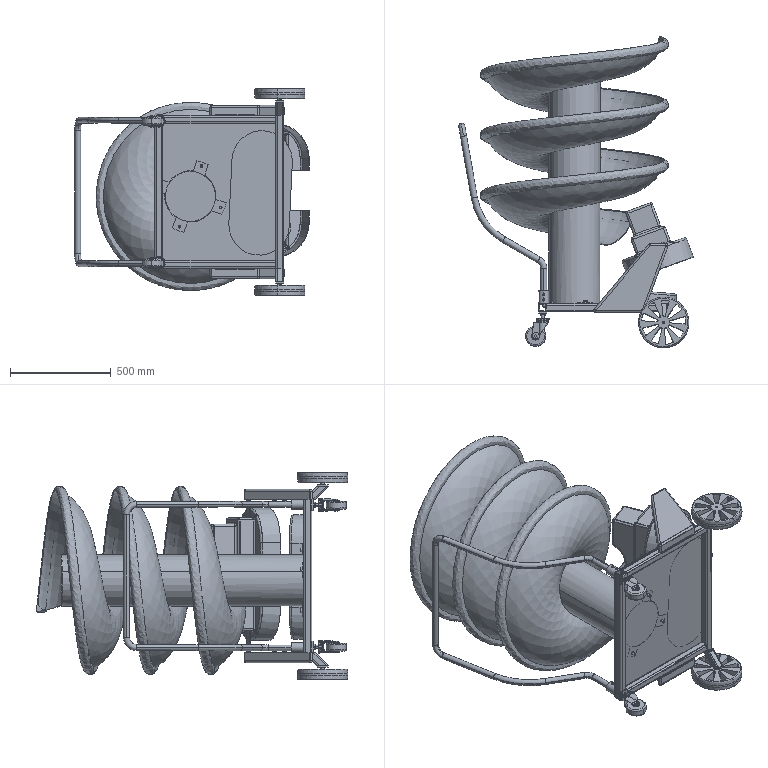Assembly | SolidWorks | mm | 43 component files | 46 solids | 1810 faces | box 1163.5 x 1546.21 x 1026 mm | volume 42101622 mm3 | cylinder 650 | plane 611 | sphere 176 | cone 160 | torus 140 | spline 73 | commonest cylinder face diameters 6 x106 20 x60 16 x50 12 x32 10 x32 14 x28 8 x24 60 x24
Bill of materials:
01-01-01ChassisWeldment1 | 1 | Q235 | Flat rectangular open frame made of four straight hollow rectangular-section tube members: two longer uprights with two shorter cross members fitted between them at the ends.
01-01-02ChassisWeldment2 | 2 | Q235 | Short length of hollow rectangular tube with rounded outer and inner corners. One end appears cut square and the other at an angle.
01-01-03ChassisWeldment3 | 2 | Q235 | Thick flat rectangular plate with rounded corners and one plain round through-hole, offset from the plate center.
01-01-04ChassisWeldment4 | 1 | Q235 | Thin flat rectangular sheet panel with four small round through-holes, spaced irregularly across the face.
01-01-05ChassisWeldment5 | 2 | 45 | Thick-walled cylindrical sleeve (bushing-like tube) with a large central bore and two small radial holes in a line along one side.
01-02WheelAxis | 2 | 45 | Stepped turned cylindrical part with a central axial bore and three diameters: a middle collar (largest), a longer upper section and a smaller lower spigot, with small chamfers at the ends.
01-03Wheel | 2 | RubberⅠ- 2 | Short disc or wheel-shaped part with a rounded outer rim, ten wedge-shaped radial cutouts forming spokes, and a small central hole.
01-04RearWheelConnectionPlate | 2 | Q235 | Flat rectangular plate with rounded corners and one round through-hole, offset toward one end.
02-01RollingTrack | 1 |  | Screw auger or helical flight: a hollow cylindrical central shaft carrying about three turns of a dished helical flight with a rolled or beaded outer edge, and small tabbed flanges with holes at one shaft end.
02-02Handrail | 1 |  | Bent round rod or tube formed into a three-dimensional U-shaped loop, with two parallel legs that each have offset joggle bends near their open ends.
03-01MotorBracket1 | 2 |  | Thin flat plate with an irregular tapered quadrilateral or pentagonal outline: a wide base edge tapering to a narrow, angled tip with a short chamfered corner.
03-02MotorBracket1 | 1 | Q235 | Long narrow flat strip with two wider square pad regions along its length. Each pad has a central round hole and four small corner holes.
03-03BallDeliveryWheel | 2 |  | Plain short solid cylinder (disc/slug) with flat parallel end faces; length is less than the diameter.
04-01MotorBracketHousing | 1 |  | Thin, flat trapezoidal plate or lid with rounded corners and edges, a solid closed top face, and several small rectangular tabs sticking out from the underside along the edges.
04-02Housing | 1 |  | Thin-walled stadium-shaped (obround) band with large rectangular gaps cut through both long sides. A stepped rectangular block projects from one side of the band, and this block has a semicircular notch cut into one edge.
04-03BottomHousing | 1 |  | Thin, flat stadium-shaped (obround) plate with a small notch in the middle of one long edge.
AC1-08M30HC0A1 | 2 |  | Box-shaped body with a square front flange, four corner through-holes, a raised circular boss in the centre of the flange, and a protruding cylindrical shaft with a flat on it. Long steps or grooves run the length of the body, and a narrower rectangular block sits at the rear. The overall shape looks like an electric motor body.
Caster-WHB31-D100-P | 2 |  | Swivel-caster-like assembly: a cylindrical wheel held in a curved single-sided fork, an axle hub with a hex nut, a round flange or washer stack on top, and a plain cylindrical stem pin pointing up.
GB_T276-94DeepGrooveBallBearing6202 | 2 | GCr4 | Open radial ball-bearing-like assembly: concentric outer and inner rings with eight spherical balls in the gap between them. No cage or shields are visible.
GB_T5781-2000HexHeadBoltFullThreadCM12x25 | 4 | 3.6 Grade | Hex-head bolt with a washer face under the head, a plain cylindrical shank and a chamfered tip.
GB_T6172.1-2000HexThinNutAAndBM16 | 2 | 04 Grade | Thin hexagonal nut with a plain cylindrical through-bore and chamfered corners on both faces.
GB_T70.1-2000_SocketHeadCapScrew_M6_16 | 2 | 8.8 Grade | Socket-head cap screw shape: a cylindrical head with a hexagonal recess, a plain cylindrical shank and a chamfered tip.
GB73-85SlottedFlatPointSetScrewM10x12 | 4 | 14H Grade | Short headless cylindrical pin with a straight slot across one end face, a small chamfer on the slotted end and a larger chamfer at the other end, similar to a slotted set screw.
Mirror04-01MotorBracketHousing | 1 |  | Shallow, open, thin-walled trapezoidal tray with rounded corners, a flat floor and small rectangular tabs standing up along the top rim.
Mates:
1. concentric | 01-02WheelAxis-1 face at (300, -53.25, 474) dir (0, 0, 1) r 6 | 01-01Chassis-1/01-01-03ChassisWeldment3-1 face at (300, -53.25, 453) dir (0, 0, 1) r 6
2. coincident | 01-01Chassis-1/01-01-03ChassisWeldment3-1 face at (314, -31.5, 453) dir (0, 0, 1) | 01-02WheelAxis-1 face at (300, -53.25, 453) dir (0, 0, -1)
3. coincident | 01-01Chassis-1 plane at (0, 0, 0) dir (0, 1, 0) | assembly plane at (0, 0, 0) dir (0, 1, 0)
4. coincident | 01-01Chassis-1 plane at (0, 0, 0) dir (0, 0, 1) | assembly plane at (0, 0, 0) dir (0, 0, 1)
5. coincident | 01-01Chassis-1 plane at (0, 0, 0) dir (1, 0, 0) | assembly plane at (0, 0, 0) dir (1, 0, 0)
6. concentric | 01-02WheelAxis-1 face at (300, -53.25, 474) dir (0, 0, 1) r 7.5 | GB_T276-94DeepGrooveBallBearing6202-2 face at (300, -53.25, 456.079) dir (0, 0, -1) r 7.5
7. coincident | 01-02WheelAxis-1 face at (300, -53.25, 463) dir (0, 0, 1) | GB_T276-94DeepGrooveBallBearing6202-2 face at (300, -42.45, 463) dir (0, 0, -1)
8. concentric | GB_T276-94DeepGrooveBallBearing6202-2 face at (300, -53.25, 468.5) dir (0, 0, -1) r 17.5 | 01-03Wheel-1 face at (300, -53.25, 474) dir (0, 0, -1) r 17.5
9. coincident | GB_T276-94DeepGrooveBallBearing6202-2 face at (300, -42.45, 474) dir (0, 0, 1) | 01-03Wheel-1 face at (300, -53.25, 474) dir (0, 0, -1)
10. concentric | 01-02WheelAxis-1 face at (300, -53.25, 474) dir (0, 0, 1) r 3 | GB_T70.1-2000_SocketHeadCapScrew_M6_16-1 face at (300, -53.25, 489) dir (0, 0, 1) r 3
11. coincident | 01-03Wheel-1 edge at (300, -53.25, 483) dir (0, 0, 1) r 4.5 | GB_T70.1-2000_SocketHeadCapScrew_M6_16-1 face at (300.832, -48.32, 483) dir (0, 0, -1)
12. coincident | 01-01Chassis-1/01-01-01ChassisWeldment1-1 face at (-312, 0, 360) dir (0, -1, 0) | 01-04RearWheelConnectionPlate-1 face at (-286, 0, 330.5) dir (0, 1, 0)
13. coincident | 01-01Chassis-1/01-01-01ChassisWeldment1-1 face at (-300, 40, 380) dir (0, 0, 1) | 01-04RearWheelConnectionPlate-1 face at (-314, 0, 380) dir (0, 0, 1)
14. coincident | 01-01Chassis-1/01-01-01ChassisWeldment1-1 face at (-320, 8, 360) dir (-1, 0, 0) | 01-04RearWheelConnectionPlate-1 face at (-320, 0, 330.5) dir (-1, 0, 0)
15. concentric | Caster-WHB31-D100-P-1 face at (-300, -171, 352.25) dir (0, -1, 0) r 8 | 01-04RearWheelConnectionPlate-1 face at (-300, 0, 352.25) dir (0, 1, 0) r 7
16. coincident | Caster-WHB31-D100-P-1 face at (-306.582, 0, 345.111) dir (0, 1, 0) | 01-04RearWheelConnectionPlate-1 face at (-286, 0, 330.5) dir (0, 1, 0)
17. concentric | Caster-WHB31-D100-P-1 face at (-300, -171, 352.25) dir (0, -1, 0) r 8 | GB_T6172.1-2000HexThinNutAAndBM16-1 face at (-300, -16, 352.25) dir (0, 1, 0) r 8
18. coincident | 01-04RearWheelConnectionPlate-1 face at (-286, -8, 330.5) dir (0, -1, 0) | GB_T6172.1-2000HexThinNutAAndBM16-1 face at (-276.834, -8, 352.25) dir (0, 1, 0)
19. parallel | 01-04RearWheelConnectionPlate-1 face at (-320, 0, 330.5) dir (-1, 0, 0) | GB_T6172.1-2000HexThinNutAAndBM16-1 face at (-311.583, -16, 358.938) dir (-1, 0, 0)
20. coincident | 01-01Chassis-1/01-01-04ChassisWeldment4-1 face at (-315, 43, 375) dir (0, 1, 0) | 02-01RollingTrack-1 face at (-142.96, 43, -22.04) dir (0, -1, 0)
21. angle | 01-01Chassis-1/01-01-01ChassisWeldment1-1 face at (300, 8, 380) dir (0, 0, 1) | 02-01RollingTrack-1 face at (-132.7, 48, 6.151) dir (0.342, 0, 0.9397)
22. coincident | 01-01Chassis-1/01-01-01ChassisWeldment1-1 face at (300, 0, 372) dir (0, -1, 0) | 03-01MotorBracket1-1 face at (-24.135, 0, 380) dir (0, -1, 0)
23. concentric | 01-01Chassis-1/01-01-05ChassisWeldment5-1 face at (-295, 103, 355) dir (0, -1, 0) r 15.1 | 02-02Handrail-1 face at (-295, 43, 355) dir (0, 1, 0) r 15
24. concentric | 01-01Chassis-1/01-01-05ChassisWeldment5-2 face at (-295, 103, -355) dir (0, -1, 0) r 15.1 | 02-02Handrail-1 face at (-295, 214.132, -355) dir (0, -1, 0) r 15
25. coincident | 01-01Chassis-1/01-01-04ChassisWeldment4-1 face at (-315, 43, 375) dir (0, 1, 0) | 02-02Handrail-1 face at (-295, 43, 355) dir (0, -1, 0)
26. concentric | 01-01Chassis-1/01-01-05ChassisWeldment5-1 face at (-295, 84, 355) dir (0, 0, -1) r 5 | GB73-85SlottedFlatPointSetScrewM10x12-1 face at (-295, 84, 382.55) dir (0, 0, 1) r 5
27. tangent | 02-02Handrail-1 face at (-295, 43, 355) dir (0, 1, 0) r 15 | GB73-85SlottedFlatPointSetScrewM10x12-1 face at (-295, 84, 370) dir (0, 0, -1)
28. coincident | 01-01Chassis-1/01-01-01ChassisWeldment1-1 face at (300, 8, 380) dir (0, 0, 1) | 03-01MotorBracket1-1 face at (-24.135, 0, 380) dir (0, 0, -1)
29. coincident | 03-01MotorBracket1-1 face at (-92.322, 187.34, 374) dir (-0.342, 0.9397, 0) | 03-02MotorBracket1-1 face at (251.015, 312.305, -1) dir (0.342, -0.9397, 0)
30. coincident | 03-01MotorBracket1-1 face at (-24.135, 0, 384) dir (0, 0, 1) | 03-02MotorBracket1-1 face at (234.57, 306.319, 384) dir (0, 0, 1)
31. coincident | 03-01MotorBracket1-1 edge at (272.158, 320, 382) dir (1, 0, 0) | 03-02MotorBracket1-1 face at (272.158, 320, 379) dir (0.9397, 0.342, 0)
32. concentric | 03-02MotorBracket1-1 face at (279.548, 326.946, 206.82) dir (-0.342, 0.9397, 0) r 2.5 | AC1-08M30HC0A1-1 face at (258.684, 384.268, 206.82) dir (-0.342, 0.9397, 0) r 3.5
33. concentric | 03-02MotorBracket1-1 face at (279.548, 326.946, 143.18) dir (-0.342, 0.9397, 0) r 2.5 | AC1-08M30HC0A1-1 face at (258.684, 384.268, 143.18) dir (-0.342, 0.9397, 0) r 3.5
34. coincident | 03-02MotorBracket1-1 face at (249.646, 316.063, -1) dir (-0.342, 0.9397, 0) | AC1-08M30HC0A1-1 face at (216.393, 303.96, 210) dir (0.342, -0.9397, 0)
35. distance | 03-03BallDeliveryWheel-1 face at (257.855, 293.511, 175) dir (-0.342, 0.9397, 0) | 03-02MotorBracket1-1 face at (251.015, 312.305, -1) dir (0.342, -0.9397, 0)
36. distance | 03-01MotorBracket1-1 edge at (-20, 4.928, 382) dir (1, 0, 0) | 01-01Chassis-1/01-01-01ChassisWeldment1-1 face at (-320, 8, 360) dir (-1, 0, 0)
37. coincident | 01-01Chassis-1/01-01-01ChassisWeldment1-1 face at (300, 8, 380) dir (0, 0, 1) | 04-01MotorBracketHousing-1 face at (-14.657, 16.888, 380) dir (0, 0, -1)
38. parallel | 03-03BallDeliveryWheel-2 face at (257.855, 293.511, -175) dir (0.342, -0.9397, 0) r 75 | 04-02Housing-1 face at (251.015, 312.305, -151.126) dir (0.342, -0.9397, 0) r 170
39. coincident | 03-02MotorBracket1-1 face at (251.015, 312.305, -1) dir (0.342, -0.9397, 0) | 04-02Housing-1 face at (251.015, 312.305, 7.874) dir (-0.342, 0.9397, 0)
40. coincident | 01-01Chassis-1/01-01-04ChassisWeldment4-1 face at (-315, 43, 375) dir (0, 1, 0) | 04-03BottomHousing-1 face at (197.547, 43, -163.468) dir (0, -1, 0)
41. coincident | 01-01Chassis-1/01-01-01ChassisWeldment1-1 face at (-320, 8, 360) dir (-1, 0, 0) | 02-01RollingTrack-1 edge at (-320, 48, 10.472) dir (0, -1, 0)
42. distance | 02-01RollingTrack-1 vertex at (-110.449, 43, 155) dir (1, 0, 0) | 01-01Chassis-1/01-01-01ChassisWeldment1-1 face at (300, 8, 380) dir (0, 0, 1)
43. concentric | 02-01RollingTrack-1 face at (-88.237, 43, 128.311) dir (0, 1, 0) r 6.75 | GB_T5781-2000HexHeadBoltFullThreadCM12x25-1 face at (-88.237, 55.5, 128.311) dir (0, 1, 0) r 6
44. coincident | 02-01RollingTrack-1 face at (-142.96, 48, -22.04) dir (0, 1, 0) | GB_T5781-2000HexHeadBoltFullThreadCM12x25-1 face at (-77.845, 48, 128.311) dir (0, -1, 0)
45. concentric | AC1-08M30HC0A1-1 face at (260.591, 285.993, 175) dir (-0.342, 0.9397, 0) r 9.5 | 03-03BallDeliveryWheel-1 face at (257.855, 293.511, 175) dir (0.342, -0.9397, 0) r 75
46. width | 04-02Housing-1 face at (208.728, 296.914, -321.126) dir (0.9397, 0.342, 0) | 04-02Housing-1 face at (293.301, 327.695, -321.126) dir (-0.9397, -0.342, 0) | 03-02MotorBracket1-1 face at (272.158, 320, 379) dir (0.9397, 0.342, 0) | 03-02MotorBracket1-1 face at (229.871, 304.609, 379) dir (-0.9397, -0.342, 0)
47. coincident | 01-01-01ChassisWeldment1-1 plane at (0, 20, 0) dir (0, 0, -1) | 01-01Chassis plane at (0, 0, 0) dir (0, 0, 1)
48. coincident | 01-01-01ChassisWeldment1-1 plane at (0, 20, 0) dir (-1, 0, 0) | 01-01Chassis plane at (0, 0, 0) dir (1, 0, 0)
49. coincident | 01-01-01ChassisWeldment1-1 face at (288, 0, 360) dir (0, -1, 0) | 01-01Chassis plane at (0, 0, 0) dir (0, 1, 0)
50. coincident | 01-01-01ChassisWeldment1-1 face at (300, 0, 380) dir (0, 0, 1) | 01-01-02ChassisWeldment2-1 face at (280, 68.222, 380) dir (0, 0, -1)
51. coincident | 01-01-01ChassisWeldment1-1 face at (312, 40, 360) dir (0, 1, 0) | 01-01-02ChassisWeldment2-1 edge at (288, 40, 380) dir (1, 0, 0)
52. coincident | 01-01-01ChassisWeldment1-1 face at (320, 32, 360) dir (1, 0, 0) | 01-01-02ChassisWeldment2-1 face at (320, 42.408, 366.279) dir (1, 0, 0)
53. coincident | 01-01-02ChassisWeldment2-1 face at (280, 68.222, 445) dir (0, 0, 1) | 01-01-03ChassisWeldment3-1 face at (314, -31.5, 445) dir (0, 0, -1)
54. distance | 01-01-03ChassisWeldment3-1 face at (286, -25.5, 453) dir (0, 1, 0) | 01-01-02ChassisWeldment2-1 edge at (312, -25, 445) dir (-1, 0, 0)
55. coincident | 01-01-02ChassisWeldment2-1 face at (320, 42.408, 366.279) dir (1, 0, 0) | 01-01-03ChassisWeldment3-1 face at (320, -31.5, 453) dir (1, 0, 0)
56. coincident | 01-01-01ChassisWeldment1-1 face at (320, 32, 360) dir (1, 0, 0) | 01-01-04ChassisWeldment4-1 face at (320, 40, 375) dir (1, 0, 0)
57. coincident | 01-01-01ChassisWeldment1-1 face at (300, 8, 380) dir (0, 0, 1) | 01-01-04ChassisWeldment4-1 edge at (-315, 43, 380) dir (1, 0, 0)
58. coincident | 01-01-01ChassisWeldment1-1 face at (-288, 40, 360) dir (0, 1, 0) | 01-01-04ChassisWeldment4-1 face at (-315, 40, 375) dir (0, -1, 0)
59. tangent | 01-01-01ChassisWeldment1-1 face at (300, 8, 380) dir (0, 0, 1) | 01-01-05ChassisWeldment5-1 face at (-295, 103, 355) dir (0, -1, 0) r 25
60. tangent | 01-01-01ChassisWeldment1-1 face at (-320, 8, 360) dir (-1, 0, 0) | 01-01-05ChassisWeldment5-1 face at (-295, 103, 355) dir (0, -1, 0) r 25
61. coincident | 01-01-04ChassisWeldment4-1 face at (-315, 43, 375) dir (0, 1, 0) | 01-01-05ChassisWeldment5-1 face at (-295, 43, 355) dir (0, -1, 0)